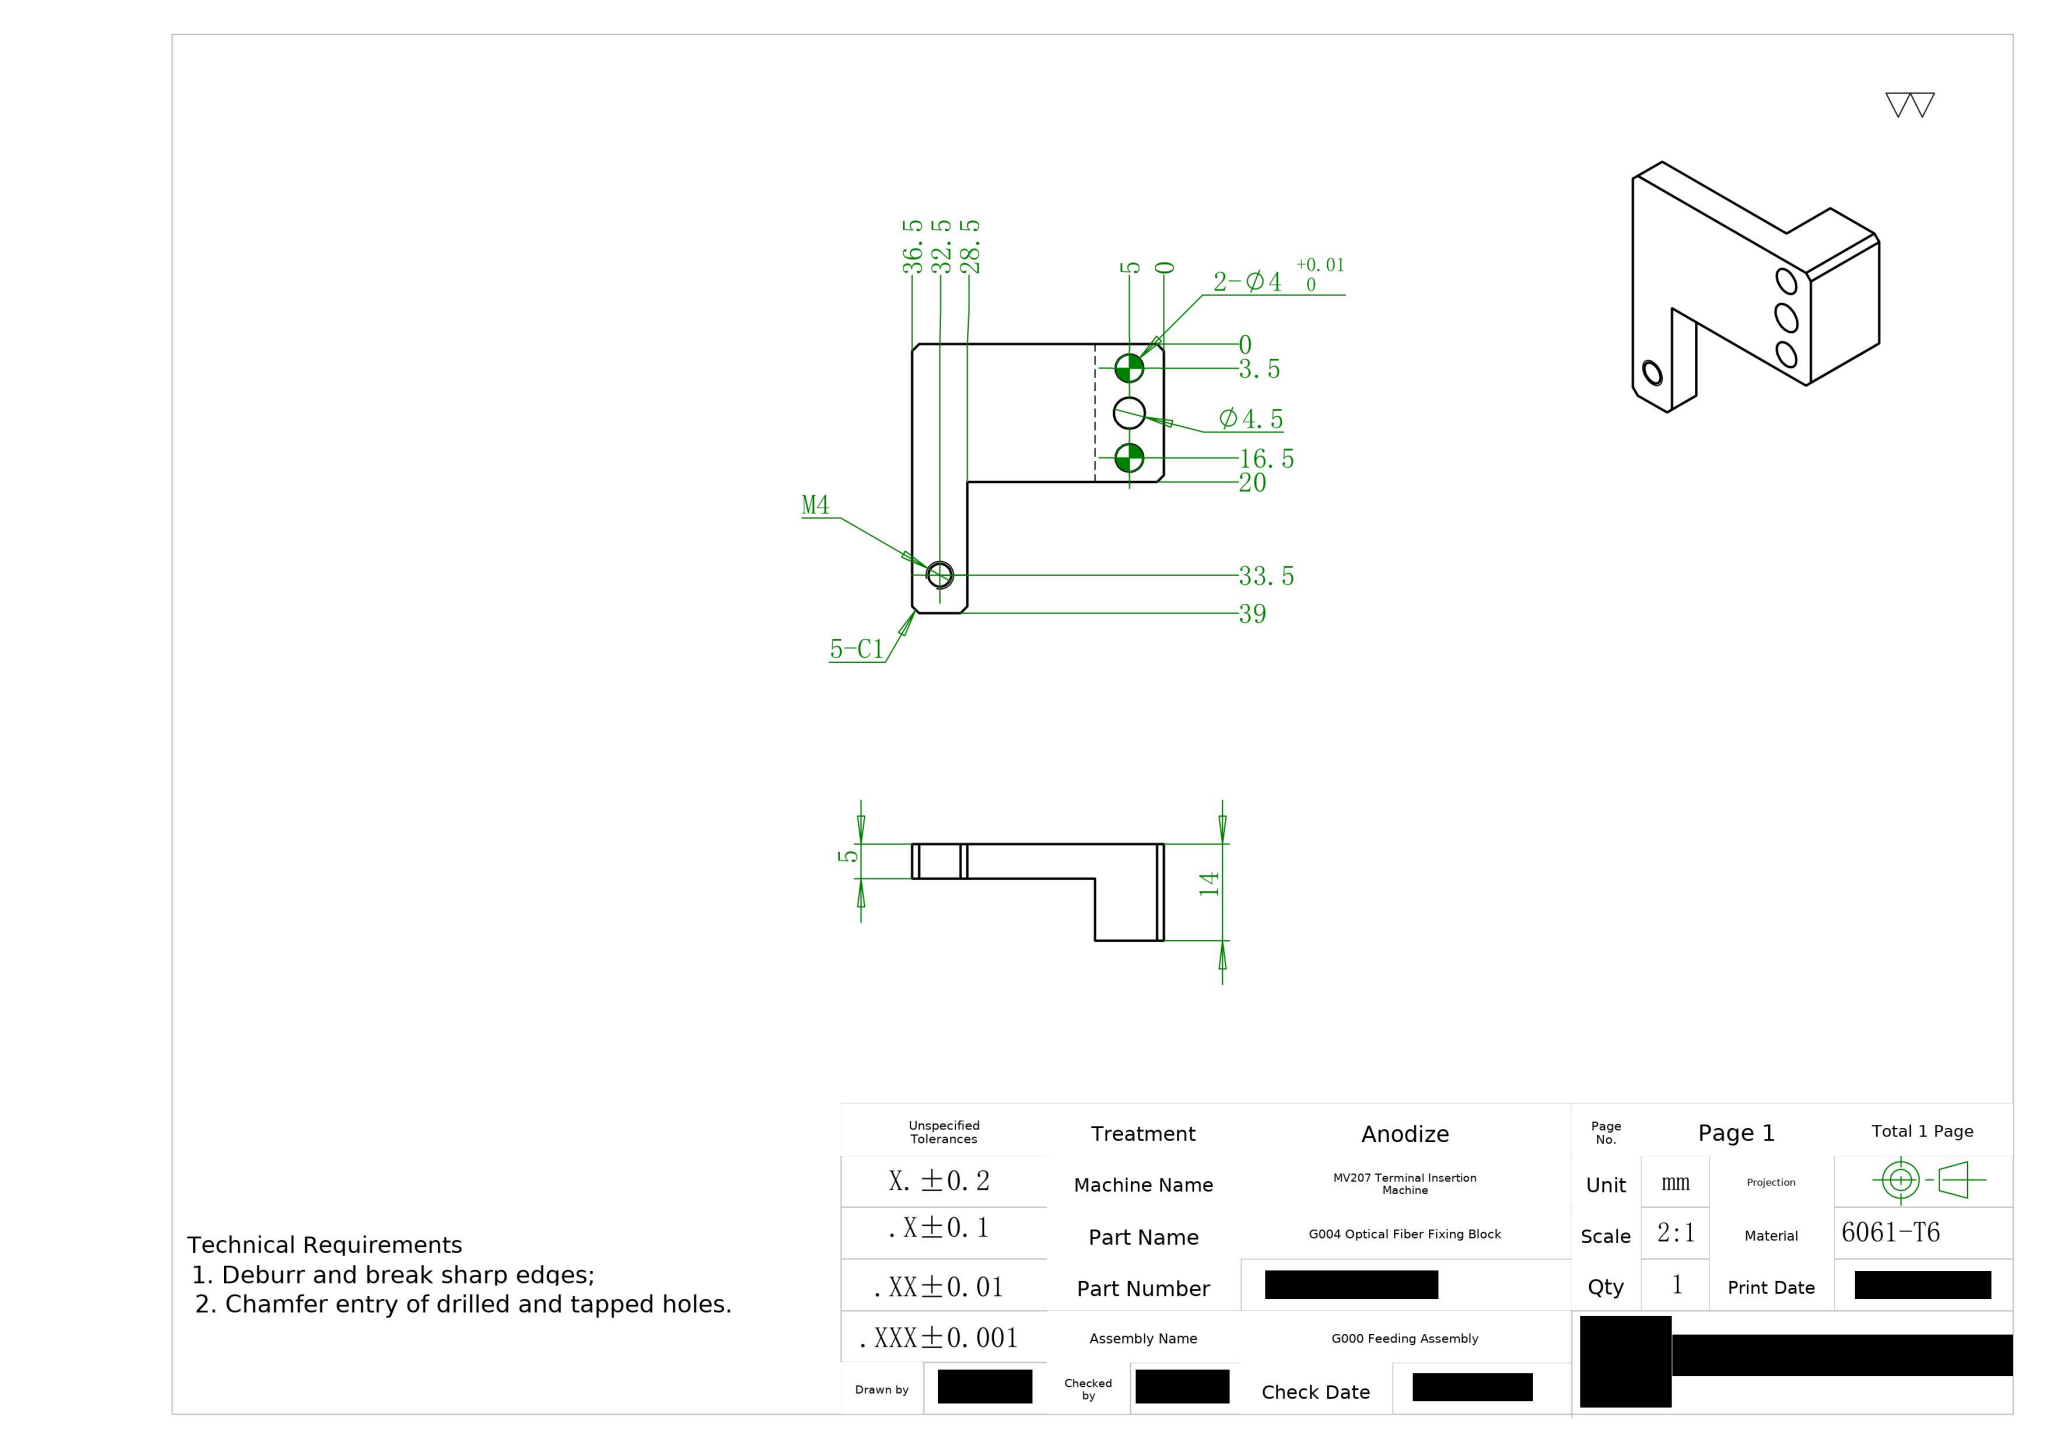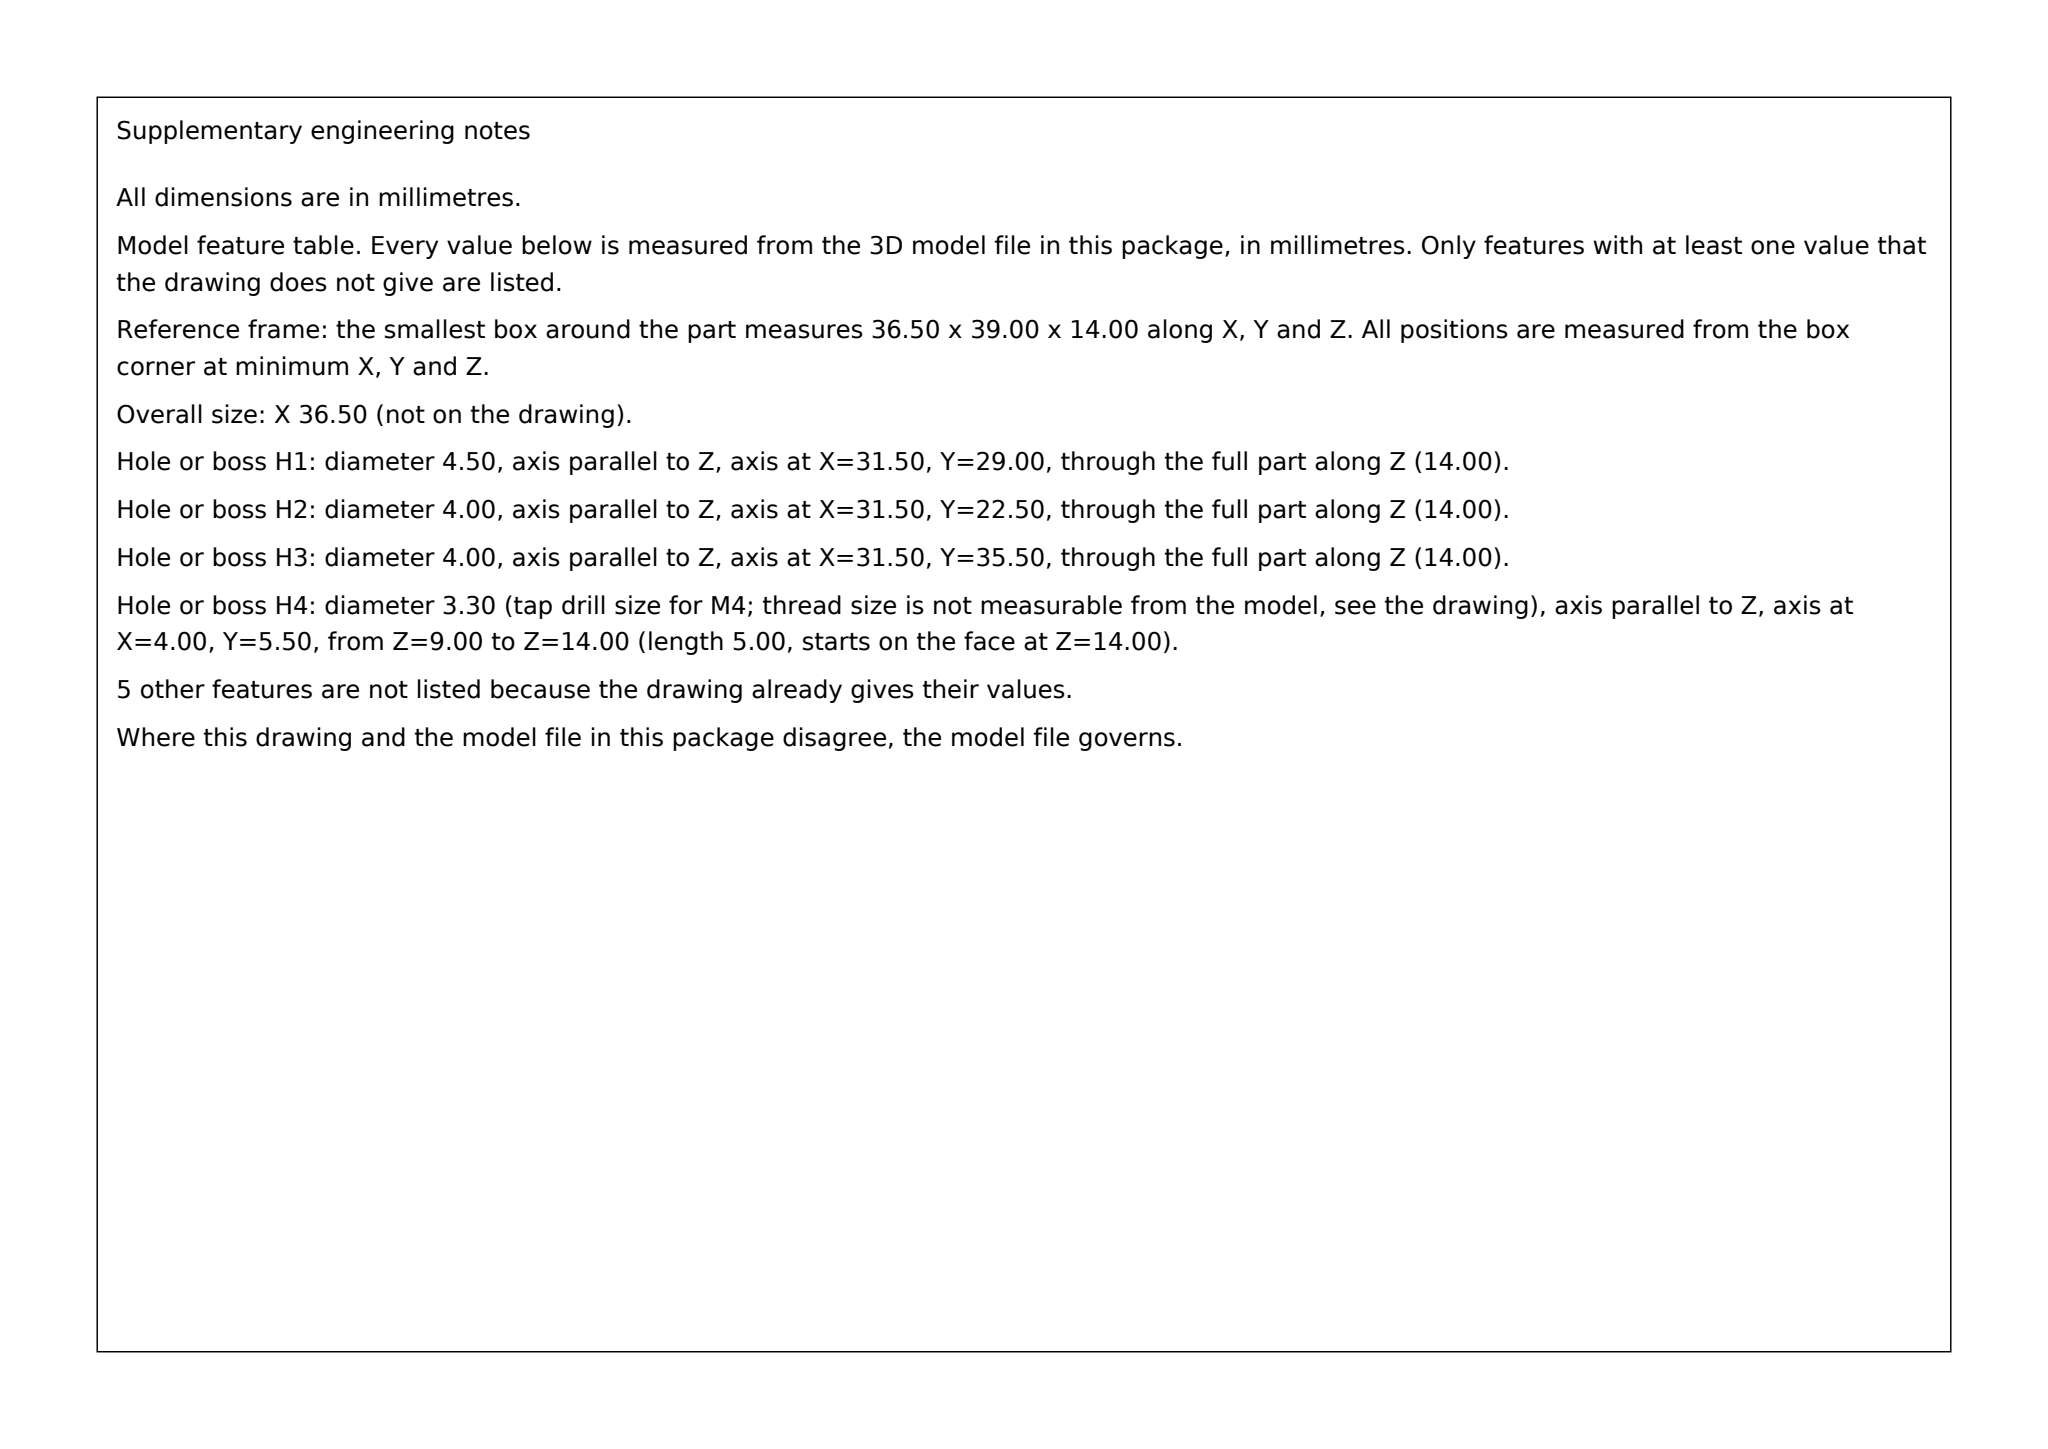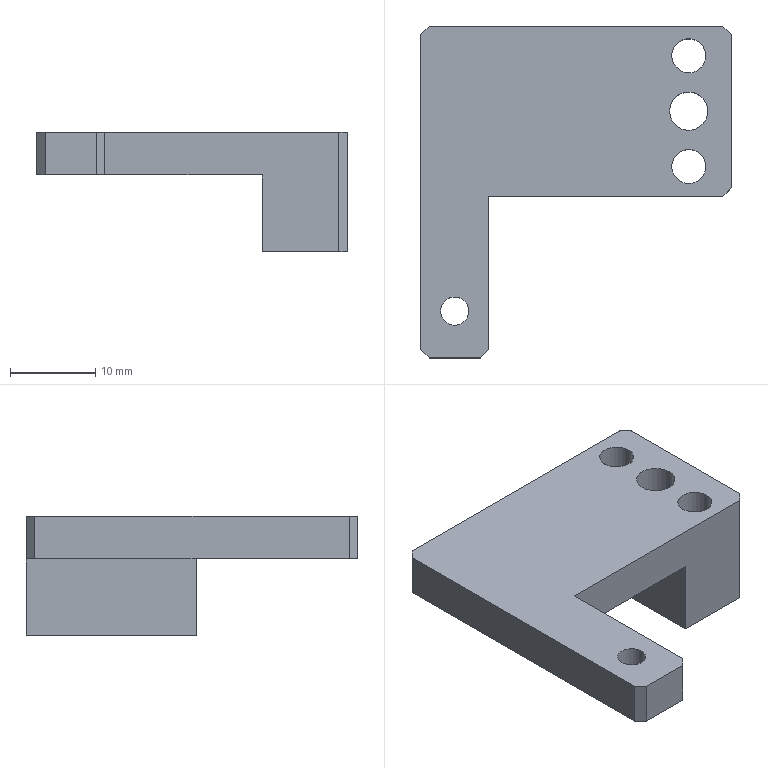Part | SolidWorks | mm | material 6061-T6 | 1 solid | 23 faces | box 36.5 x 39 x 14 mm | volume 5571 mm3 | plane 15 | cylinder 8 | commonest cylinder face diameters 4 x4 4.5 x2 3.3 x2
build123d program:
from build123d import *

# Parameters (mm, degrees)
SKETCH1_W                  = 36.5
SKETCH1_H                  = 11
BOSS_EXTRUDE1_DEPTH        = 5
M4_TAPPED_HOLE1_D          = 3.3
SKETCH4_W                  = 9.5
SKETCH4_H                  = 28
BOSS_EXTRUDE2_DEPTH        = 5
SKETCH5_W                  = 5
SKETCH5_H                  = 28
BOSS_EXTRUDE3_DEPTH        = 27
SKETCH6_W                  = 28.5
SKETCH6_H                  = 19
CUT_EXTRUDE1_DEPTH         = 39.475
SKETCH9_W                  = 10
SKETCH9_H                  = 20
BOSS_EXTRUDE4_DEPTH        = 9
F_4_0_4_DIAMETER_HOLE1_D   = 4
CHAMFER1_SIZE              = 1
F_4_5_4_5_DIAMETER_HOLE1_D = 4.5


with BuildPart() as part:
    # Sketch1 → Boss-Extrude1 (new body)
    with BuildSketch(Plane.XY):
        Rectangle(SKETCH1_W, SKETCH1_H)
    extrude(amount=BOSS_EXTRUDE1_DEPTH)

    # M4 Tapped Hole1 (through all)
    with Locations(Plane.XY.offset(5)):
        with Locations((-14.25, 0)):
            Hole(M4_TAPPED_HOLE1_D / 2)

    # Sketch4 → Boss-Extrude2 (add)
    with BuildSketch(Plane.XY.offset(5)):
        with Locations((13.5, 19.5)):
            Rectangle(SKETCH4_W, SKETCH4_H)
    extrude(amount=-BOSS_EXTRUDE2_DEPTH)

    # Sketch5 → Boss-Extrude3 (add)
    with BuildSketch(Plane.ZY.offset(-8.75)):
        with Locations((2.5, 19.5)):
            Rectangle(SKETCH5_W, SKETCH5_H)
    extrude(amount=BOSS_EXTRUDE3_DEPTH)

    # Sketch6 → Cut-Extrude1 (cut, through all)
    with BuildSketch(Plane.XY.offset(5)):
        with Locations((4, 4)):
            Rectangle(SKETCH6_W, SKETCH6_H)
    extrude(amount=-CUT_EXTRUDE1_DEPTH, mode=Mode.SUBTRACT)

    # Sketch9 → Boss-Extrude4 (add)
    with BuildSketch(Plane(origin=(0, 0, 0), x_dir=(-1, 0, 0), z_dir=(0, 0, -1))):
        with Locations((-13.25, 23.5)):
            Rectangle(SKETCH9_W, SKETCH9_H)
    extrude(amount=BOSS_EXTRUDE4_DEPTH)

    # 4.0 _4_ Diameter Hole1 (through all)
    with Locations(Plane.XY.offset(5)):
        with Locations((13.25, 17), (13.25, 30)):
            Hole(F_4_0_4_DIAMETER_HOLE1_D / 2)

    # Chamfer1
    chamfer1_edges = [part.edges().sort_by_distance(p)[0] for p in [
        (18.25, 33.5, -2),
        (-18.25, 33.5, 2.5),
        (18.25, 13.5, -2),
        (-10.25, -5.5, 2.5),
        (-18.25, -5.5, 2.5),
    ]]
    chamfer(chamfer1_edges, length=CHAMFER1_SIZE)

    # 4.5 _4.5_ Diameter Hole1 (through all)
    with Locations(Plane.XY.offset(5)):
        with Locations((13.25, 23.5)):
            Hole(F_4_5_4_5_DIAMETER_HOLE1_D / 2)


solid = part.part
STEP:
#1=CARTESIAN_POINT('',(11.,23.5,-9.));
#2=VERTEX_POINT('',#1);
#3=CARTESIAN_POINT('',(15.5,23.5,-9.));
#4=VERTEX_POINT('',#3);
#5=CARTESIAN_POINT('',(13.25,23.5,-9.));
#6=DIRECTION('',(0.,0.,1.));
#7=DIRECTION('',(1.,0.,0.));
#8=AXIS2_PLACEMENT_3D('',#5,#6,#7);
#9=CIRCLE('',#8,2.25);
#10=EDGE_CURVE('',#2,#4,#9,.T.);
#11=ORIENTED_EDGE('',*,*,#10,.F.);
#12=CARTESIAN_POINT('',(11.,23.5,5.));
#13=VERTEX_POINT('',#12);
#14=CARTESIAN_POINT('',(11.,23.5,5.));
#15=DIRECTION('',(0.,0.,1.));
#16=VECTOR('',#15,1000.);
#17=LINE('',#14,#16);
#18=EDGE_CURVE('',#2,#13,#17,.T.);
#19=ORIENTED_EDGE('',*,*,#18,.T.);
#20=CARTESIAN_POINT('',(15.5,23.5,5.));
#21=VERTEX_POINT('',#20);
#22=CARTESIAN_POINT('',(13.25,23.5,5.));
#23=DIRECTION('',(0.,0.,1.));
#24=DIRECTION('',(1.,0.,0.));
#25=AXIS2_PLACEMENT_3D('',#22,#23,#24);
#26=CIRCLE('',#25,2.25);
#27=EDGE_CURVE('',#13,#21,#26,.T.);
#28=ORIENTED_EDGE('',*,*,#27,.T.);
#29=CARTESIAN_POINT('',(15.5,23.5,5.));
#30=DIRECTION('',(0.,0.,1.));
#31=VECTOR('',#30,1000.);
#32=LINE('',#29,#31);
#33=EDGE_CURVE('',#4,#21,#32,.T.);
#34=ORIENTED_EDGE('',*,*,#33,.F.);
#35=EDGE_LOOP('',(#11,#19,#28,#34));
#36=FACE_OUTER_BOUND('',#35,.T.);
#37=CARTESIAN_POINT('',(13.25,23.5,5.));
#38=DIRECTION('',(0.,0.,1.));
#39=DIRECTION('',(1.,0.,0.));
#40=AXIS2_PLACEMENT_3D('',#37,#38,#39);
#41=CYLINDRICAL_SURFACE('',#40,2.25);
#42=ADVANCED_FACE('',(#36),#41,.F.);
#43=CARTESIAN_POINT('',(11.25,17.,-9.));
#44=VERTEX_POINT('',#43);
#45=CARTESIAN_POINT('',(15.25,17.,-9.));
#46=VERTEX_POINT('',#45);
#47=CARTESIAN_POINT('',(13.25,17.,-9.));
#48=DIRECTION('',(0.,0.,1.));
#49=DIRECTION('',(1.,0.,0.));
#50=AXIS2_PLACEMENT_3D('',#47,#48,#49);
#51=CIRCLE('',#50,2.);
#52=EDGE_CURVE('',#44,#46,#51,.T.);
#53=ORIENTED_EDGE('',*,*,#52,.F.);
#54=CARTESIAN_POINT('',(11.25,17.,5.));
#55=VERTEX_POINT('',#54);
#56=CARTESIAN_POINT('',(11.25,17.,5.));
#57=DIRECTION('',(0.,0.,1.));
#58=VECTOR('',#57,1000.);
#59=LINE('',#56,#58);
#60=EDGE_CURVE('',#44,#55,#59,.T.);
#61=ORIENTED_EDGE('',*,*,#60,.T.);
#62=CARTESIAN_POINT('',(15.25,17.,5.));
#63=VERTEX_POINT('',#62);
#64=CARTESIAN_POINT('',(13.25,17.,5.));
#65=DIRECTION('',(0.,0.,1.));
#66=DIRECTION('',(1.,0.,0.));
#67=AXIS2_PLACEMENT_3D('',#64,#65,#66);
#68=CIRCLE('',#67,2.);
#69=EDGE_CURVE('',#55,#63,#68,.T.);
#70=ORIENTED_EDGE('',*,*,#69,.T.);
#71=CARTESIAN_POINT('',(15.25,17.,5.));
#72=DIRECTION('',(0.,0.,1.));
#73=VECTOR('',#72,1000.);
#74=LINE('',#71,#73);
#75=EDGE_CURVE('',#46,#63,#74,.T.);
#76=ORIENTED_EDGE('',*,*,#75,.F.);
#77=EDGE_LOOP('',(#53,#61,#70,#76));
#78=FACE_OUTER_BOUND('',#77,.T.);
#79=CARTESIAN_POINT('',(13.25,17.,5.));
#80=DIRECTION('',(0.,0.,1.));
#81=DIRECTION('',(1.,0.,0.));
#82=AXIS2_PLACEMENT_3D('',#79,#80,#81);
#83=CYLINDRICAL_SURFACE('',#82,2.);
#84=ADVANCED_FACE('',(#78),#83,.F.);
#85=CARTESIAN_POINT('',(11.25,30.,-9.));
#86=VERTEX_POINT('',#85);
#87=CARTESIAN_POINT('',(15.25,30.,-9.));
#88=VERTEX_POINT('',#87);
#89=CARTESIAN_POINT('',(13.25,30.,-9.));
#90=DIRECTION('',(0.,0.,1.));
#91=DIRECTION('',(1.,0.,0.));
#92=AXIS2_PLACEMENT_3D('',#89,#90,#91);
#93=CIRCLE('',#92,2.);
#94=EDGE_CURVE('',#86,#88,#93,.T.);
#95=ORIENTED_EDGE('',*,*,#94,.F.);
#96=CARTESIAN_POINT('',(11.25,30.,5.));
#97=VERTEX_POINT('',#96);
#98=CARTESIAN_POINT('',(11.25,30.,5.));
#99=DIRECTION('',(0.,0.,1.));
#100=VECTOR('',#99,1000.);
#101=LINE('',#98,#100);
#102=EDGE_CURVE('',#86,#97,#101,.T.);
#103=ORIENTED_EDGE('',*,*,#102,.T.);
#104=CARTESIAN_POINT('',(15.25,30.,5.));
#105=VERTEX_POINT('',#104);
#106=CARTESIAN_POINT('',(13.25,30.,5.));
#107=DIRECTION('',(0.,0.,1.));
#108=DIRECTION('',(1.,0.,0.));
#109=AXIS2_PLACEMENT_3D('',#106,#107,#108);
#110=CIRCLE('',#109,2.);
#111=EDGE_CURVE('',#97,#105,#110,.T.);
#112=ORIENTED_EDGE('',*,*,#111,.T.);
#113=CARTESIAN_POINT('',(15.25,30.,5.));
#114=DIRECTION('',(0.,0.,1.));
#115=VECTOR('',#114,1000.);
#116=LINE('',#113,#115);
#117=EDGE_CURVE('',#88,#105,#116,.T.);
#118=ORIENTED_EDGE('',*,*,#117,.F.);
#119=EDGE_LOOP('',(#95,#103,#112,#118));
#120=FACE_OUTER_BOUND('',#119,.T.);
#121=CARTESIAN_POINT('',(13.25,30.,5.));
#122=DIRECTION('',(0.,0.,1.));
#123=DIRECTION('',(1.,0.,0.));
#124=AXIS2_PLACEMENT_3D('',#121,#122,#123);
#125=CYLINDRICAL_SURFACE('',#124,2.);
#126=ADVANCED_FACE('',(#120),#125,.F.);
#127=CARTESIAN_POINT('',(-15.9,-0.,0.));
#128=VERTEX_POINT('',#127);
#129=CARTESIAN_POINT('',(-12.6,-0.,0.));
#130=VERTEX_POINT('',#129);
#131=CARTESIAN_POINT('',(-14.25,-0.,0.));
#132=DIRECTION('',(0.,0.,1.));
#133=DIRECTION('',(1.,0.,0.));
#134=AXIS2_PLACEMENT_3D('',#131,#132,#133);
#135=CIRCLE('',#134,1.65);
#136=EDGE_CURVE('',#128,#130,#135,.T.);
#137=ORIENTED_EDGE('',*,*,#136,.F.);
#138=CARTESIAN_POINT('',(-15.9,-0.,5.));
#139=VERTEX_POINT('',#138);
#140=CARTESIAN_POINT('',(-15.9,-0.,5.));
#141=DIRECTION('',(0.,0.,1.));
#142=VECTOR('',#141,1000.);
#143=LINE('',#140,#142);
#144=EDGE_CURVE('',#128,#139,#143,.T.);
#145=ORIENTED_EDGE('',*,*,#144,.T.);
#146=CARTESIAN_POINT('',(-12.6,-0.,5.));
#147=VERTEX_POINT('',#146);
#148=CARTESIAN_POINT('',(-14.25,-0.,5.));
#149=DIRECTION('',(0.,0.,1.));
#150=DIRECTION('',(1.,0.,0.));
#151=AXIS2_PLACEMENT_3D('',#148,#149,#150);
#152=CIRCLE('',#151,1.65);
#153=EDGE_CURVE('',#139,#147,#152,.T.);
#154=ORIENTED_EDGE('',*,*,#153,.T.);
#155=CARTESIAN_POINT('',(-12.6,-0.,5.));
#156=DIRECTION('',(0.,0.,1.));
#157=VECTOR('',#156,1000.);
#158=LINE('',#155,#157);
#159=EDGE_CURVE('',#130,#147,#158,.T.);
#160=ORIENTED_EDGE('',*,*,#159,.F.);
#161=EDGE_LOOP('',(#137,#145,#154,#160));
#162=FACE_OUTER_BOUND('',#161,.T.);
#163=CARTESIAN_POINT('',(-14.25,-0.,5.));
#164=DIRECTION('',(0.,0.,1.));
#165=DIRECTION('',(1.,0.,0.));
#166=AXIS2_PLACEMENT_3D('',#163,#164,#165);
#167=CYLINDRICAL_SURFACE('',#166,1.65);
#168=ADVANCED_FACE('',(#162),#167,.F.);
#169=CARTESIAN_POINT('',(-14.25,-0.,0.));
#170=DIRECTION('',(0.,0.,1.));
#171=DIRECTION('',(1.,0.,0.));
#172=AXIS2_PLACEMENT_3D('',#169,#170,#171);
#173=CIRCLE('',#172,1.65);
#174=EDGE_CURVE('',#130,#128,#173,.T.);
#175=ORIENTED_EDGE('',*,*,#174,.T.);
#176=ORIENTED_EDGE('',*,*,#136,.T.);
#177=EDGE_LOOP('',(#175,#176));
#178=FACE_BOUND('',#177,.T.);
#179=CARTESIAN_POINT('',(-10.25,13.5,0.));
#180=VERTEX_POINT('',#179);
#181=CARTESIAN_POINT('',(-10.25,-4.5,0.));
#182=VERTEX_POINT('',#181);
#183=CARTESIAN_POINT('',(-10.25,-5.5,0.));
#184=DIRECTION('',(0.,-1.,0.));
#185=VECTOR('',#184,1000.);
#186=LINE('',#183,#185);
#187=EDGE_CURVE('',#180,#182,#186,.T.);
#188=ORIENTED_EDGE('',*,*,#187,.T.);
#189=CARTESIAN_POINT('',(-11.25,-5.5,0.));
#190=VERTEX_POINT('',#189);
#191=CARTESIAN_POINT('',(-11.25,-5.5,0.));
#192=DIRECTION('',(-0.7071,-0.7071,0.));
#193=VECTOR('',#192,1000.);
#194=LINE('',#191,#193);
#195=EDGE_CURVE('',#182,#190,#194,.T.);
#196=ORIENTED_EDGE('',*,*,#195,.T.);
#197=CARTESIAN_POINT('',(-17.25,-5.5,0.));
#198=VERTEX_POINT('',#197);
#199=CARTESIAN_POINT('',(-18.25,-5.5,0.));
#200=DIRECTION('',(1.,0.,0.));
#201=VECTOR('',#200,1000.);
#202=LINE('',#199,#201);
#203=EDGE_CURVE('',#198,#190,#202,.T.);
#204=ORIENTED_EDGE('',*,*,#203,.F.);
#205=CARTESIAN_POINT('',(-18.25,-4.5,0.));
#206=VERTEX_POINT('',#205);
#207=CARTESIAN_POINT('',(-17.25,-5.5,0.));
#208=DIRECTION('',(-0.7071,0.7071,0.));
#209=VECTOR('',#208,1000.);
#210=LINE('',#207,#209);
#211=EDGE_CURVE('',#198,#206,#210,.T.);
#212=ORIENTED_EDGE('',*,*,#211,.T.);
#213=CARTESIAN_POINT('',(-18.25,32.5,0.));
#214=VERTEX_POINT('',#213);
#215=CARTESIAN_POINT('',(-18.25,5.5,0.));
#216=DIRECTION('',(0.,-1.,0.));
#217=VECTOR('',#216,1000.);
#218=LINE('',#215,#217);
#219=EDGE_CURVE('',#214,#206,#218,.T.);
#220=ORIENTED_EDGE('',*,*,#219,.F.);
#221=CARTESIAN_POINT('',(-17.25,33.5,0.));
#222=VERTEX_POINT('',#221);
#223=CARTESIAN_POINT('',(-17.25,33.5,0.));
#224=DIRECTION('',(0.7071,0.7071,0.));
#225=VECTOR('',#224,1000.);
#226=LINE('',#223,#225);
#227=EDGE_CURVE('',#214,#222,#226,.T.);
#228=ORIENTED_EDGE('',*,*,#227,.T.);
#229=CARTESIAN_POINT('',(8.25,33.5,0.));
#230=VERTEX_POINT('',#229);
#231=CARTESIAN_POINT('',(18.25,33.5,0.));
#232=DIRECTION('',(-1.,0.,0.));
#233=VECTOR('',#232,1000.);
#234=LINE('',#231,#233);
#235=EDGE_CURVE('',#230,#222,#234,.T.);
#236=ORIENTED_EDGE('',*,*,#235,.F.);
#237=CARTESIAN_POINT('',(8.25,13.5,0.));
#238=VERTEX_POINT('',#237);
#239=CARTESIAN_POINT('',(8.25,13.5,0.));
#240=DIRECTION('',(0.,1.,0.));
#241=VECTOR('',#240,1000.);
#242=LINE('',#239,#241);
#243=EDGE_CURVE('',#238,#230,#242,.T.);
#244=ORIENTED_EDGE('',*,*,#243,.F.);
#245=CARTESIAN_POINT('',(18.25,13.5,0.));
#246=DIRECTION('',(-1.,-0.,0.));
#247=VECTOR('',#246,1000.);
#248=LINE('',#245,#247);
#249=EDGE_CURVE('',#238,#180,#248,.T.);
#250=ORIENTED_EDGE('',*,*,#249,.T.);
#251=EDGE_LOOP('',(#188,#196,#204,#212,#220,#228,#236,#244,#250));
#252=FACE_OUTER_BOUND('',#251,.T.);
#253=CARTESIAN_POINT('',(0.,0.,0.));
#254=DIRECTION('',(0.,0.,1.));
#255=DIRECTION('',(1.,0.,0.));
#256=AXIS2_PLACEMENT_3D('',#253,#254,#255);
#257=PLANE('',#256);
#258=ADVANCED_FACE('',(#178,#252),#257,.F.);
#259=CARTESIAN_POINT('',(18.25,14.5,5.));
#260=VERTEX_POINT('',#259);
#261=CARTESIAN_POINT('',(18.25,32.5,5.));
#262=VERTEX_POINT('',#261);
#263=CARTESIAN_POINT('',(18.25,5.5,5.));
#264=DIRECTION('',(0.,1.,0.));
#265=VECTOR('',#264,1000.);
#266=LINE('',#263,#265);
#267=EDGE_CURVE('',#260,#262,#266,.T.);
#268=ORIENTED_EDGE('',*,*,#267,.F.);
#269=CARTESIAN_POINT('',(18.25,14.5,-9.));
#270=VERTEX_POINT('',#269);
#271=CARTESIAN_POINT('',(18.25,14.5,5.));
#272=DIRECTION('',(0.,0.,-1.));
#273=VECTOR('',#272,1000.);
#274=LINE('',#271,#273);
#275=EDGE_CURVE('',#260,#270,#274,.T.);
#276=ORIENTED_EDGE('',*,*,#275,.T.);
#277=CARTESIAN_POINT('',(18.25,32.5,-9.));
#278=VERTEX_POINT('',#277);
#279=CARTESIAN_POINT('',(18.25,13.5,-9.));
#280=DIRECTION('',(0.,-1.,0.));
#281=VECTOR('',#280,1000.);
#282=LINE('',#279,#281);
#283=EDGE_CURVE('',#278,#270,#282,.T.);
#284=ORIENTED_EDGE('',*,*,#283,.F.);
#285=CARTESIAN_POINT('',(18.25,32.5,5.));
#286=DIRECTION('',(0.,0.,1.));
#287=VECTOR('',#286,1000.);
#288=LINE('',#285,#287);
#289=EDGE_CURVE('',#278,#262,#288,.T.);
#290=ORIENTED_EDGE('',*,*,#289,.T.);
#291=EDGE_LOOP('',(#268,#276,#284,#290));
#292=FACE_OUTER_BOUND('',#291,.T.);
#293=CARTESIAN_POINT('',(18.25,5.5,5.));
#294=DIRECTION('',(-1.,0.,0.));
#295=DIRECTION('',(0.,0.,1.));
#296=AXIS2_PLACEMENT_3D('',#293,#294,#295);
#297=PLANE('',#296);
#298=ADVANCED_FACE('',(#292),#297,.F.);
#299=ORIENTED_EDGE('',*,*,#219,.T.);
#300=CARTESIAN_POINT('',(-18.25,-4.5,5.));
#301=VERTEX_POINT('',#300);
#302=CARTESIAN_POINT('',(-18.25,-4.5,5.));
#303=DIRECTION('',(0.,0.,1.));
#304=VECTOR('',#303,1000.);
#305=LINE('',#302,#304);
#306=EDGE_CURVE('',#206,#301,#305,.T.);
#307=ORIENTED_EDGE('',*,*,#306,.T.);
#308=CARTESIAN_POINT('',(-18.25,32.5,5.));
#309=VERTEX_POINT('',#308);
#310=CARTESIAN_POINT('',(-18.25,5.5,5.));
#311=DIRECTION('',(0.,-1.,0.));
#312=VECTOR('',#311,1000.);
#313=LINE('',#310,#312);
#314=EDGE_CURVE('',#309,#301,#313,.T.);
#315=ORIENTED_EDGE('',*,*,#314,.F.);
#316=CARTESIAN_POINT('',(-18.25,32.5,0.));
#317=DIRECTION('',(0.,0.,-1.));
#318=VECTOR('',#317,1000.);
#319=LINE('',#316,#318);
#320=EDGE_CURVE('',#309,#214,#319,.T.);
#321=ORIENTED_EDGE('',*,*,#320,.T.);
#322=EDGE_LOOP('',(#299,#307,#315,#321));
#323=FACE_OUTER_BOUND('',#322,.T.);
#324=CARTESIAN_POINT('',(-18.25,5.5,5.));
#325=DIRECTION('',(1.,0.,0.));
#326=DIRECTION('',(0.,0.,-1.));
#327=AXIS2_PLACEMENT_3D('',#324,#325,#326);
#328=PLANE('',#327);
#329=ADVANCED_FACE('',(#323),#328,.F.);
#330=ORIENTED_EDGE('',*,*,#203,.T.);
#331=CARTESIAN_POINT('',(-11.25,-5.5,5.));
#332=VERTEX_POINT('',#331);
#333=CARTESIAN_POINT('',(-11.25,-5.5,5.));
#334=DIRECTION('',(0.,0.,1.));
#335=VECTOR('',#334,1000.);
#336=LINE('',#333,#335);
#337=EDGE_CURVE('',#190,#332,#336,.T.);
#338=ORIENTED_EDGE('',*,*,#337,.T.);
#339=CARTESIAN_POINT('',(-17.25,-5.5,5.));
#340=VERTEX_POINT('',#339);
#341=CARTESIAN_POINT('',(-18.25,-5.5,5.));
#342=DIRECTION('',(1.,0.,0.));
#343=VECTOR('',#342,1000.);
#344=LINE('',#341,#343);
#345=EDGE_CURVE('',#340,#332,#344,.T.);
#346=ORIENTED_EDGE('',*,*,#345,.F.);
#347=CARTESIAN_POINT('',(-17.25,-5.5,5.));
#348=DIRECTION('',(0.,0.,-1.));
#349=VECTOR('',#348,1000.);
#350=LINE('',#347,#349);
#351=EDGE_CURVE('',#340,#198,#350,.T.);
#352=ORIENTED_EDGE('',*,*,#351,.T.);
#353=EDGE_LOOP('',(#330,#338,#346,#352));
#354=FACE_OUTER_BOUND('',#353,.T.);
#355=CARTESIAN_POINT('',(-18.25,-5.5,5.));
#356=DIRECTION('',(0.,1.,0.));
#357=DIRECTION('',(0.,0.,1.));
#358=AXIS2_PLACEMENT_3D('',#355,#356,#357);
#359=PLANE('',#358);
#360=ADVANCED_FACE('',(#354),#359,.F.);
#361=CARTESIAN_POINT('',(13.25,23.5,5.));
#362=DIRECTION('',(0.,0.,1.));
#363=DIRECTION('',(1.,0.,0.));
#364=AXIS2_PLACEMENT_3D('',#361,#362,#363);
#365=CIRCLE('',#364,2.25);
#366=EDGE_CURVE('',#21,#13,#365,.T.);
#367=ORIENTED_EDGE('',*,*,#366,.F.);
#368=ORIENTED_EDGE('',*,*,#27,.F.);
#369=EDGE_LOOP('',(#367,#368));
#370=FACE_BOUND('',#369,.T.);
#371=CARTESIAN_POINT('',(13.25,17.,5.));
#372=DIRECTION('',(0.,0.,1.));
#373=DIRECTION('',(1.,0.,0.));
#374=AXIS2_PLACEMENT_3D('',#371,#372,#373);
#375=CIRCLE('',#374,2.);
#376=EDGE_CURVE('',#63,#55,#375,.T.);
#377=ORIENTED_EDGE('',*,*,#376,.F.);
#378=ORIENTED_EDGE('',*,*,#69,.F.);
#379=EDGE_LOOP('',(#377,#378));
#380=FACE_BOUND('',#379,.T.);
#381=CARTESIAN_POINT('',(13.25,30.,5.));
#382=DIRECTION('',(0.,0.,1.));
#383=DIRECTION('',(1.,0.,0.));
#384=AXIS2_PLACEMENT_3D('',#381,#382,#383);
#385=CIRCLE('',#384,2.);
#386=EDGE_CURVE('',#105,#97,#385,.T.);
#387=ORIENTED_EDGE('',*,*,#386,.F.);
#388=ORIENTED_EDGE('',*,*,#111,.F.);
#389=EDGE_LOOP('',(#387,#388));
#390=FACE_BOUND('',#389,.T.);
#391=CARTESIAN_POINT('',(17.25,13.5,5.));
#392=VERTEX_POINT('',#391);
#393=CARTESIAN_POINT('',(-10.25,13.5,5.));
#394=VERTEX_POINT('',#393);
#395=CARTESIAN_POINT('',(18.25,13.5,5.));
#396=DIRECTION('',(-1.,-0.,0.));
#397=VECTOR('',#396,1000.);
#398=LINE('',#395,#397);
#399=EDGE_CURVE('',#392,#394,#398,.T.);
#400=ORIENTED_EDGE('',*,*,#399,.F.);
#401=CARTESIAN_POINT('',(1.875,-1.875,5.));
#402=DIRECTION('',(0.7071,0.7071,0.));
#403=VECTOR('',#402,1000.);
#404=LINE('',#401,#403);
#405=EDGE_CURVE('',#392,#260,#404,.T.);
#406=ORIENTED_EDGE('',*,*,#405,.T.);
#407=ORIENTED_EDGE('',*,*,#267,.T.);
#408=CARTESIAN_POINT('',(17.25,33.5,5.));
#409=VERTEX_POINT('',#408);
#410=CARTESIAN_POINT('',(25.375,25.375,5.));
#411=DIRECTION('',(-0.7071,0.7071,0.));
#412=VECTOR('',#411,1000.);
#413=LINE('',#410,#412);
#414=EDGE_CURVE('',#262,#409,#413,.T.);
#415=ORIENTED_EDGE('',*,*,#414,.T.);
#416=CARTESIAN_POINT('',(-17.25,33.5,5.));
#417=VERTEX_POINT('',#416);
#418=CARTESIAN_POINT('',(18.25,33.5,5.));
#419=DIRECTION('',(-1.,0.,0.));
#420=VECTOR('',#419,1000.);
#421=LINE('',#418,#420);
#422=EDGE_CURVE('',#409,#417,#421,.T.);
#423=ORIENTED_EDGE('',*,*,#422,.T.);
#424=CARTESIAN_POINT('',(-25.375,25.375,5.));
#425=DIRECTION('',(-0.7071,-0.7071,0.));
#426=VECTOR('',#425,1000.);
#427=LINE('',#424,#426);
#428=EDGE_CURVE('',#417,#309,#427,.T.);
#429=ORIENTED_EDGE('',*,*,#428,.T.);
#430=ORIENTED_EDGE('',*,*,#314,.T.);
#431=CARTESIAN_POINT('',(-11.375,-11.375,5.));
#432=DIRECTION('',(0.7071,-0.7071,0.));
#433=VECTOR('',#432,1000.);
#434=LINE('',#431,#433);
#435=EDGE_CURVE('',#301,#340,#434,.T.);
#436=ORIENTED_EDGE('',*,*,#435,.T.);
#437=ORIENTED_EDGE('',*,*,#345,.T.);
#438=CARTESIAN_POINT('',(-10.25,-4.5,5.));
#439=VERTEX_POINT('',#438);
#440=CARTESIAN_POINT('',(-2.875,2.875,5.));
#441=DIRECTION('',(0.7071,0.7071,0.));
#442=VECTOR('',#441,1000.);
#443=LINE('',#440,#442);
#444=EDGE_CURVE('',#332,#439,#443,.T.);
#445=ORIENTED_EDGE('',*,*,#444,.T.);
#446=CARTESIAN_POINT('',(-10.25,-5.5,5.));
#447=DIRECTION('',(0.,-1.,0.));
#448=VECTOR('',#447,1000.);
#449=LINE('',#446,#448);
#450=EDGE_CURVE('',#394,#439,#449,.T.);
#451=ORIENTED_EDGE('',*,*,#450,.F.);
#452=EDGE_LOOP('',(#400,#406,#407,#415,#423,#429,#430,#436,#437,#445,#451));
#453=FACE_OUTER_BOUND('',#452,.T.);
#454=CARTESIAN_POINT('',(-14.25,-0.,5.));
#455=DIRECTION('',(0.,0.,1.));
#456=DIRECTION('',(1.,0.,0.));
#457=AXIS2_PLACEMENT_3D('',#454,#455,#456);
#458=CIRCLE('',#457,1.65);
#459=EDGE_CURVE('',#147,#139,#458,.T.);
#460=ORIENTED_EDGE('',*,*,#459,.F.);
#461=ORIENTED_EDGE('',*,*,#153,.F.);
#462=EDGE_LOOP('',(#460,#461));
#463=FACE_BOUND('',#462,.T.);
#464=CARTESIAN_POINT('',(0.,0.,5.));
#465=DIRECTION('',(0.,0.,1.));
#466=DIRECTION('',(1.,0.,0.));
#467=AXIS2_PLACEMENT_3D('',#464,#465,#466);
#468=PLANE('',#467);
#469=ADVANCED_FACE('',(#370,#380,#390,#453,#463),#468,.T.);
#470=ORIENTED_EDGE('',*,*,#144,.F.);
#471=ORIENTED_EDGE('',*,*,#174,.F.);
#472=ORIENTED_EDGE('',*,*,#159,.T.);
#473=ORIENTED_EDGE('',*,*,#459,.T.);
#474=EDGE_LOOP('',(#470,#471,#472,#473));
#475=FACE_OUTER_BOUND('',#474,.T.);
#476=CARTESIAN_POINT('',(-14.25,-0.,5.));
#477=DIRECTION('',(0.,0.,1.));
#478=DIRECTION('',(1.,0.,0.));
#479=AXIS2_PLACEMENT_3D('',#476,#477,#478);
#480=CYLINDRICAL_SURFACE('',#479,1.65);
#481=ADVANCED_FACE('',(#475),#480,.F.);
#482=ORIENTED_EDGE('',*,*,#422,.F.);
#483=CARTESIAN_POINT('',(17.25,33.5,-9.));
#484=VERTEX_POINT('',#483);
#485=CARTESIAN_POINT('',(17.25,33.5,-9.));
#486=DIRECTION('',(0.,0.,-1.));
#487=VECTOR('',#486,1000.);
#488=LINE('',#485,#487);
#489=EDGE_CURVE('',#409,#484,#488,.T.);
#490=ORIENTED_EDGE('',*,*,#489,.T.);
#491=CARTESIAN_POINT('',(8.25,33.5,-9.));
#492=VERTEX_POINT('',#491);
#493=CARTESIAN_POINT('',(18.25,33.5,-9.));
#494=DIRECTION('',(1.,0.,0.));
#495=VECTOR('',#494,1000.);
#496=LINE('',#493,#495);
#497=EDGE_CURVE('',#492,#484,#496,.T.);
#498=ORIENTED_EDGE('',*,*,#497,.F.);
#499=CARTESIAN_POINT('',(8.25,33.5,-9.));
#500=DIRECTION('',(0.,0.,1.));
#501=VECTOR('',#500,1000.);
#502=LINE('',#499,#501);
#503=EDGE_CURVE('',#492,#230,#502,.T.);
#504=ORIENTED_EDGE('',*,*,#503,.T.);
#505=ORIENTED_EDGE('',*,*,#235,.T.);
#506=CARTESIAN_POINT('',(-17.25,33.5,5.));
#507=DIRECTION('',(0.,0.,1.));
#508=VECTOR('',#507,1000.);
#509=LINE('',#506,#508);
#510=EDGE_CURVE('',#222,#417,#509,.T.);
#511=ORIENTED_EDGE('',*,*,#510,.T.);
#512=EDGE_LOOP('',(#482,#490,#498,#504,#505,#511));
#513=FACE_OUTER_BOUND('',#512,.T.);
#514=CARTESIAN_POINT('',(18.25,33.5,0.));
#515=DIRECTION('',(0.,1.,0.));
#516=DIRECTION('',(0.,0.,1.));
#517=AXIS2_PLACEMENT_3D('',#514,#515,#516);
#518=PLANE('',#517);
#519=ADVANCED_FACE('',(#513),#518,.T.);
#520=ORIENTED_EDGE('',*,*,#450,.T.);
#521=CARTESIAN_POINT('',(-10.25,-4.5,0.));
#522=DIRECTION('',(0.,0.,-1.));
#523=VECTOR('',#522,1000.);
#524=LINE('',#521,#523);
#525=EDGE_CURVE('',#439,#182,#524,.T.);
#526=ORIENTED_EDGE('',*,*,#525,.T.);
#527=ORIENTED_EDGE('',*,*,#187,.F.);
#528=CARTESIAN_POINT('',(-10.25,13.5,0.));
#529=DIRECTION('',(0.,0.,1.));
#530=VECTOR('',#529,1000.);
#531=LINE('',#528,#530);
#532=EDGE_CURVE('',#180,#394,#531,.T.);
#533=ORIENTED_EDGE('',*,*,#532,.T.);
#534=EDGE_LOOP('',(#520,#526,#527,#533));
#535=FACE_OUTER_BOUND('',#534,.T.);
#536=CARTESIAN_POINT('',(-10.25,-5.5,0.));
#537=DIRECTION('',(-1.,0.,0.));
#538=DIRECTION('',(0.,0.,1.));
#539=AXIS2_PLACEMENT_3D('',#536,#537,#538);
#540=PLANE('',#539);
#541=ADVANCED_FACE('',(#535),#540,.F.);
#542=CARTESIAN_POINT('',(17.25,13.5,-9.));
#543=VERTEX_POINT('',#542);
#544=CARTESIAN_POINT('',(8.25,13.5,-9.));
#545=VERTEX_POINT('',#544);
#546=CARTESIAN_POINT('',(18.25,13.5,-9.));
#547=DIRECTION('',(-1.,0.,0.));
#548=VECTOR('',#547,1000.);
#549=LINE('',#546,#548);
#550=EDGE_CURVE('',#543,#545,#549,.T.);
#551=ORIENTED_EDGE('',*,*,#550,.F.);
#552=CARTESIAN_POINT('',(17.25,13.5,0.));
#553=DIRECTION('',(0.,0.,1.));
#554=VECTOR('',#553,1000.);
#555=LINE('',#552,#554);
#556=EDGE_CURVE('',#543,#392,#555,.T.);
#557=ORIENTED_EDGE('',*,*,#556,.T.);
#558=ORIENTED_EDGE('',*,*,#399,.T.);
#559=ORIENTED_EDGE('',*,*,#532,.F.);
#560=ORIENTED_EDGE('',*,*,#249,.F.);
#561=CARTESIAN_POINT('',(8.25,13.5,-9.));
#562=DIRECTION('',(0.,0.,1.));
#563=VECTOR('',#562,1000.);
#564=LINE('',#561,#563);
#565=EDGE_CURVE('',#545,#238,#564,.T.);
#566=ORIENTED_EDGE('',*,*,#565,.F.);
#567=EDGE_LOOP('',(#551,#557,#558,#559,#560,#566));
#568=FACE_OUTER_BOUND('',#567,.T.);
#569=CARTESIAN_POINT('',(18.25,13.5,0.));
#570=DIRECTION('',(-0.,1.,0.));
#571=DIRECTION('',(-1.,-0.,0.));
#572=AXIS2_PLACEMENT_3D('',#569,#570,#571);
#573=PLANE('',#572);
#574=ADVANCED_FACE('',(#568),#573,.F.);
#575=ORIENTED_EDGE('',*,*,#243,.T.);
#576=ORIENTED_EDGE('',*,*,#503,.F.);
#577=CARTESIAN_POINT('',(8.25,13.5,-9.));
#578=DIRECTION('',(0.,1.,0.));
#579=VECTOR('',#578,1000.);
#580=LINE('',#577,#579);
#581=EDGE_CURVE('',#545,#492,#580,.T.);
#582=ORIENTED_EDGE('',*,*,#581,.F.);
#583=ORIENTED_EDGE('',*,*,#565,.T.);
#584=EDGE_LOOP('',(#575,#576,#582,#583));
#585=FACE_OUTER_BOUND('',#584,.T.);
#586=CARTESIAN_POINT('',(8.25,13.5,-9.));
#587=DIRECTION('',(1.,0.,0.));
#588=DIRECTION('',(0.,0.,-1.));
#589=AXIS2_PLACEMENT_3D('',#586,#587,#588);
#590=PLANE('',#589);
#591=ADVANCED_FACE('',(#585),#590,.F.);
#592=CARTESIAN_POINT('',(13.25,23.5,-9.));
#593=DIRECTION('',(0.,0.,1.));
#594=DIRECTION('',(1.,0.,0.));
#595=AXIS2_PLACEMENT_3D('',#592,#593,#594);
#596=CIRCLE('',#595,2.25);
#597=EDGE_CURVE('',#4,#2,#596,.T.);
#598=ORIENTED_EDGE('',*,*,#597,.T.);
#599=ORIENTED_EDGE('',*,*,#10,.T.);
#600=EDGE_LOOP('',(#598,#599));
#601=FACE_BOUND('',#600,.T.);
#602=CARTESIAN_POINT('',(13.25,17.,-9.));
#603=DIRECTION('',(0.,0.,1.));
#604=DIRECTION('',(1.,0.,0.));
#605=AXIS2_PLACEMENT_3D('',#602,#603,#604);
#606=CIRCLE('',#605,2.);
#607=EDGE_CURVE('',#46,#44,#606,.T.);
#608=ORIENTED_EDGE('',*,*,#607,.T.);
#609=ORIENTED_EDGE('',*,*,#52,.T.);
#610=EDGE_LOOP('',(#608,#609));
#611=FACE_BOUND('',#610,.T.);
#612=CARTESIAN_POINT('',(13.25,30.,-9.));
#613=DIRECTION('',(0.,0.,1.));
#614=DIRECTION('',(1.,0.,0.));
#615=AXIS2_PLACEMENT_3D('',#612,#613,#614);
#616=CIRCLE('',#615,2.);
#617=EDGE_CURVE('',#88,#86,#616,.T.);
#618=ORIENTED_EDGE('',*,*,#617,.T.);
#619=ORIENTED_EDGE('',*,*,#94,.T.);
#620=EDGE_LOOP('',(#618,#619));
#621=FACE_BOUND('',#620,.T.);
#622=ORIENTED_EDGE('',*,*,#283,.T.);
#623=CARTESIAN_POINT('',(17.25,13.5,-9.));
#624=DIRECTION('',(-0.7071,-0.7071,0.));
#625=VECTOR('',#624,1000.);
#626=LINE('',#623,#625);
#627=EDGE_CURVE('',#270,#543,#626,.T.);
#628=ORIENTED_EDGE('',*,*,#627,.T.);
#629=ORIENTED_EDGE('',*,*,#550,.T.);
#630=ORIENTED_EDGE('',*,*,#581,.T.);
#631=ORIENTED_EDGE('',*,*,#497,.T.);
#632=CARTESIAN_POINT('',(18.25,32.5,-9.));
#633=DIRECTION('',(0.7071,-0.7071,0.));
#634=VECTOR('',#633,1000.);
#635=LINE('',#632,#634);
#636=EDGE_CURVE('',#484,#278,#635,.T.);
#637=ORIENTED_EDGE('',*,*,#636,.T.);
#638=EDGE_LOOP('',(#622,#628,#629,#630,#631,#637));
#639=FACE_OUTER_BOUND('',#638,.T.);
#640=CARTESIAN_POINT('',(0.,0.,-9.));
#641=DIRECTION('',(0.,0.,1.));
#642=DIRECTION('',(1.,0.,0.));
#643=AXIS2_PLACEMENT_3D('',#640,#641,#642);
#644=PLANE('',#643);
#645=ADVANCED_FACE('',(#601,#611,#621,#639),#644,.F.);
#646=ORIENTED_EDGE('',*,*,#102,.F.);
#647=ORIENTED_EDGE('',*,*,#617,.F.);
#648=ORIENTED_EDGE('',*,*,#117,.T.);
#649=ORIENTED_EDGE('',*,*,#386,.T.);
#650=EDGE_LOOP('',(#646,#647,#648,#649));
#651=FACE_OUTER_BOUND('',#650,.T.);
#652=CARTESIAN_POINT('',(13.25,30.,5.));
#653=DIRECTION('',(0.,0.,1.));
#654=DIRECTION('',(1.,0.,0.));
#655=AXIS2_PLACEMENT_3D('',#652,#653,#654);
#656=CYLINDRICAL_SURFACE('',#655,2.);
#657=ADVANCED_FACE('',(#651),#656,.F.);
#658=ORIENTED_EDGE('',*,*,#60,.F.);
#659=ORIENTED_EDGE('',*,*,#607,.F.);
#660=ORIENTED_EDGE('',*,*,#75,.T.);
#661=ORIENTED_EDGE('',*,*,#376,.T.);
#662=EDGE_LOOP('',(#658,#659,#660,#661));
#663=FACE_OUTER_BOUND('',#662,.T.);
#664=CARTESIAN_POINT('',(13.25,17.,5.));
#665=DIRECTION('',(0.,0.,1.));
#666=DIRECTION('',(1.,0.,0.));
#667=AXIS2_PLACEMENT_3D('',#664,#665,#666);
#668=CYLINDRICAL_SURFACE('',#667,2.);
#669=ADVANCED_FACE('',(#663),#668,.F.);
#670=ORIENTED_EDGE('',*,*,#627,.F.);
#671=ORIENTED_EDGE('',*,*,#275,.F.);
#672=ORIENTED_EDGE('',*,*,#405,.F.);
#673=ORIENTED_EDGE('',*,*,#556,.F.);
#674=EDGE_LOOP('',(#670,#671,#672,#673));
#675=FACE_OUTER_BOUND('',#674,.T.);
#676=CARTESIAN_POINT('',(17.25,13.5,0.));
#677=DIRECTION('',(-0.7071,0.7071,0.));
#678=DIRECTION('',(0.,0.,1.));
#679=AXIS2_PLACEMENT_3D('',#676,#677,#678);
#680=PLANE('',#679);
#681=ADVANCED_FACE('',(#675),#680,.F.);
#682=ORIENTED_EDGE('',*,*,#636,.F.);
#683=ORIENTED_EDGE('',*,*,#489,.F.);
#684=ORIENTED_EDGE('',*,*,#414,.F.);
#685=ORIENTED_EDGE('',*,*,#289,.F.);
#686=EDGE_LOOP('',(#682,#683,#684,#685));
#687=FACE_OUTER_BOUND('',#686,.T.);
#688=CARTESIAN_POINT('',(18.25,32.5,5.));
#689=DIRECTION('',(0.7071,0.7071,0.));
#690=DIRECTION('',(0.,0.,-1.));
#691=AXIS2_PLACEMENT_3D('',#688,#689,#690);
#692=PLANE('',#691);
#693=ADVANCED_FACE('',(#687),#692,.T.);
#694=ORIENTED_EDGE('',*,*,#195,.F.);
#695=ORIENTED_EDGE('',*,*,#525,.F.);
#696=ORIENTED_EDGE('',*,*,#444,.F.);
#697=ORIENTED_EDGE('',*,*,#337,.F.);
#698=EDGE_LOOP('',(#694,#695,#696,#697));
#699=FACE_OUTER_BOUND('',#698,.T.);
#700=CARTESIAN_POINT('',(-11.25,-5.5,5.));
#701=DIRECTION('',(-0.7071,0.7071,0.));
#702=DIRECTION('',(0.,0.,1.));
#703=AXIS2_PLACEMENT_3D('',#700,#701,#702);
#704=PLANE('',#703);
#705=ADVANCED_FACE('',(#699),#704,.F.);
#706=ORIENTED_EDGE('',*,*,#435,.F.);
#707=ORIENTED_EDGE('',*,*,#306,.F.);
#708=ORIENTED_EDGE('',*,*,#211,.F.);
#709=ORIENTED_EDGE('',*,*,#351,.F.);
#710=EDGE_LOOP('',(#706,#707,#708,#709));
#711=FACE_OUTER_BOUND('',#710,.T.);
#712=CARTESIAN_POINT('',(-17.25,-5.5,5.));
#713=DIRECTION('',(0.7071,0.7071,0.));
#714=DIRECTION('',(0.,0.,-1.));
#715=AXIS2_PLACEMENT_3D('',#712,#713,#714);
#716=PLANE('',#715);
#717=ADVANCED_FACE('',(#711),#716,.F.);
#718=ORIENTED_EDGE('',*,*,#227,.F.);
#719=ORIENTED_EDGE('',*,*,#320,.F.);
#720=ORIENTED_EDGE('',*,*,#428,.F.);
#721=ORIENTED_EDGE('',*,*,#510,.F.);
#722=EDGE_LOOP('',(#718,#719,#720,#721));
#723=FACE_OUTER_BOUND('',#722,.T.);
#724=CARTESIAN_POINT('',(-17.25,33.5,0.));
#725=DIRECTION('',(-0.7071,0.7071,0.));
#726=DIRECTION('',(0.,0.,-1.));
#727=AXIS2_PLACEMENT_3D('',#724,#725,#726);
#728=PLANE('',#727);
#729=ADVANCED_FACE('',(#723),#728,.T.);
#730=ORIENTED_EDGE('',*,*,#18,.F.);
#731=ORIENTED_EDGE('',*,*,#597,.F.);
#732=ORIENTED_EDGE('',*,*,#33,.T.);
#733=ORIENTED_EDGE('',*,*,#366,.T.);
#734=EDGE_LOOP('',(#730,#731,#732,#733));
#735=FACE_OUTER_BOUND('',#734,.T.);
#736=CARTESIAN_POINT('',(13.25,23.5,5.));
#737=DIRECTION('',(0.,0.,1.));
#738=DIRECTION('',(1.,0.,0.));
#739=AXIS2_PLACEMENT_3D('',#736,#737,#738);
#740=CYLINDRICAL_SURFACE('',#739,2.25);
#741=ADVANCED_FACE('',(#735),#740,.F.);
#742=CLOSED_SHELL('',(#42,#84,#126,#168,#258,#298,#329,#360,#469,#481,#519,#541,#574,#591,#645,#657,#669,#681,#693,#705,#717,#729,#741));
#743=MANIFOLD_SOLID_BREP('',#742);
#744=CARTESIAN_POINT('',(0.,0.,0.));
#745=DIRECTION('',(0.,0.,1.));
#746=DIRECTION('',(1.,0.,0.));
#747=AXIS2_PLACEMENT_3D('',#744,#745,#746);
#748=(LENGTH_UNIT()NAMED_UNIT(*)SI_UNIT(.MILLI.,.METRE.));
#749=UNCERTAINTY_MEASURE_WITH_UNIT(LENGTH_MEASURE(0.00001),#748,'','');
#750=(NAMED_UNIT(*)PLANE_ANGLE_UNIT()SI_UNIT($,.RADIAN.));
#751=(NAMED_UNIT(*)SI_UNIT($,.STERADIAN.)SOLID_ANGLE_UNIT());
#752=(GEOMETRIC_REPRESENTATION_CONTEXT(3)GLOBAL_UNCERTAINTY_ASSIGNED_CONTEXT((#749))GLOBAL_UNIT_ASSIGNED_CONTEXT((#748,#750,#751))REPRESENTATION_CONTEXT('',''));
#753=ADVANCED_BREP_SHAPE_REPRESENTATION('',(#743,#747),#752);